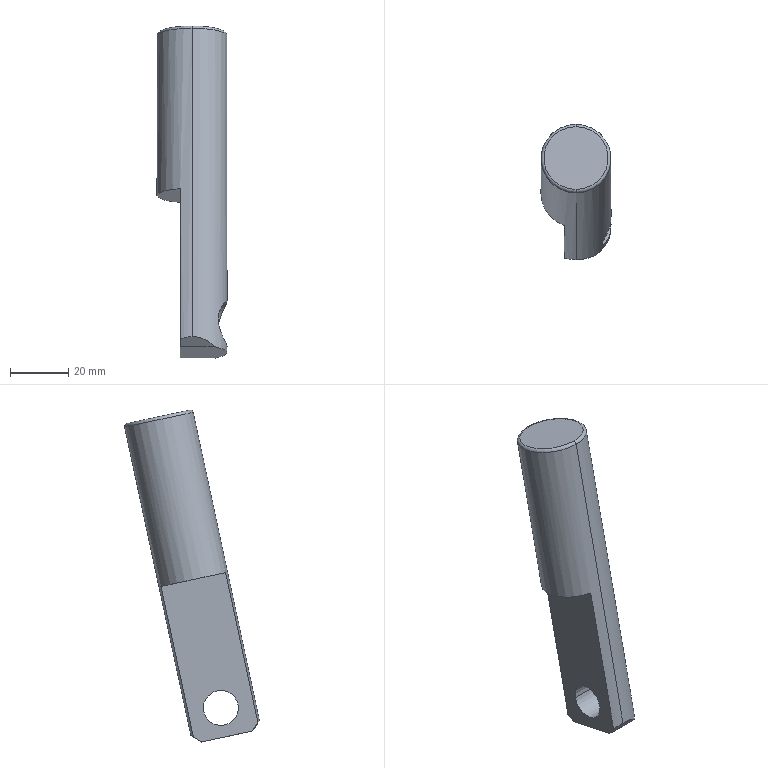Component | SolidWorks | SwingRod-2 | 1 solid | 15 faces | box 24 x 46.18 x 113.72 mm | volume 41126 mm3 | plane 7 | cylinder 6 | torus 2 | commonest cylinder face diameters 16 x2 12 x2 24 x2
STEP:
#1=COLOUR_RGB('',0.7922,0.8196,0.9333);
#2=FILL_AREA_STYLE_COLOUR('',#1);
#3=FILL_AREA_STYLE('',(#2));
#4=SURFACE_STYLE_FILL_AREA(#3);
#5=SURFACE_SIDE_STYLE('',(#4));
#6=SURFACE_STYLE_USAGE(.BOTH.,#5);
#7=PRESENTATION_STYLE_ASSIGNMENT((#6));
#8=CARTESIAN_POINT('',(6.39,3.505,17.411));
#9=VERTEX_POINT('',#8);
#10=CARTESIAN_POINT('',(6.39,2.658,17.593));
#11=VERTEX_POINT('',#10);
#12=CARTESIAN_POINT('',(6.39,3.081,17.502));
#13=DIRECTION('',(0.,0.2101,0.9777));
#14=DIRECTION('',(0.,-0.9777,0.2101));
#15=AXIS2_PLACEMENT_3D('',#12,#13,#14);
#16=CIRCLE('',#15,0.4331);
#17=EDGE_CURVE('',#9,#11,#16,.T.);
#18=ORIENTED_EDGE('',*,*,#17,.F.);
#19=CARTESIAN_POINT('',(6.39,3.535,17.365));
#20=VERTEX_POINT('',#19);
#21=CARTESIAN_POINT('',(6.39,3.496,17.373));
#22=DIRECTION('',(-1.,0.,0.));
#23=DIRECTION('',(0.,0.,1.));
#24=AXIS2_PLACEMENT_3D('',#21,#22,#23);
#25=CIRCLE('',#24,0.03937);
#26=EDGE_CURVE('',#9,#20,#25,.T.);
#27=ORIENTED_EDGE('',*,*,#26,.T.);
#28=CARTESIAN_POINT('',(6.39,2.611,17.563));
#29=VERTEX_POINT('',#28);
#30=CARTESIAN_POINT('',(6.39,3.073,17.464));
#31=DIRECTION('',(-0.,-0.2101,-0.9777));
#32=DIRECTION('',(0.,-0.9777,0.2101));
#33=AXIS2_PLACEMENT_3D('',#30,#31,#32);
#34=CIRCLE('',#33,0.4724);
#35=EDGE_CURVE('',#29,#20,#34,.T.);
#36=ORIENTED_EDGE('',*,*,#35,.F.);
#37=CARTESIAN_POINT('',(6.39,2.65,17.555));
#38=DIRECTION('',(1.,-0.,-0.));
#39=DIRECTION('',(-0.,0.,-1.));
#40=AXIS2_PLACEMENT_3D('',#37,#38,#39);
#41=CIRCLE('',#40,0.03937);
#42=EDGE_CURVE('',#11,#29,#41,.T.);
#43=ORIENTED_EDGE('',*,*,#42,.F.);
#44=EDGE_LOOP('',(#18,#27,#36,#43));
#45=FACE_OUTER_BOUND('',#44,.T.);
#46=CARTESIAN_POINT('',(6.39,3.073,17.464));
#47=DIRECTION('',(-0.,-0.2101,-0.9777));
#48=DIRECTION('',(0.,-0.9777,0.2101));
#49=AXIS2_PLACEMENT_3D('',#46,#47,#48);
#50=TOROIDAL_SURFACE('',#49,0.4331,0.03937);
#51=ADVANCED_FACE('',(#45),#50,.T.);
#52=CARTESIAN_POINT('',(6.742,2.546,13.51));
#53=VERTEX_POINT('',#52);
#54=CARTESIAN_POINT('',(6.742,1.93,13.642));
#55=VERTEX_POINT('',#54);
#56=CARTESIAN_POINT('',(6.742,2.546,13.51));
#57=CARTESIAN_POINT('',(6.742,2.55,13.531));
#58=CARTESIAN_POINT('',(6.744,2.552,13.552));
#59=CARTESIAN_POINT('',(6.749,2.553,13.584));
#60=CARTESIAN_POINT('',(6.751,2.552,13.594));
#61=CARTESIAN_POINT('',(6.757,2.55,13.615));
#62=CARTESIAN_POINT('',(6.759,2.549,13.625));
#63=CARTESIAN_POINT('',(6.766,2.545,13.645));
#64=CARTESIAN_POINT('',(6.769,2.543,13.655));
#65=CARTESIAN_POINT('',(6.776,2.537,13.674));
#66=CARTESIAN_POINT('',(6.779,2.534,13.684));
#67=CARTESIAN_POINT('',(6.791,2.523,13.712));
#68=CARTESIAN_POINT('',(6.798,2.514,13.73));
#69=CARTESIAN_POINT('',(6.813,2.492,13.763));
#70=CARTESIAN_POINT('',(6.821,2.479,13.779));
#71=CARTESIAN_POINT('',(6.834,2.452,13.808));
#72=CARTESIAN_POINT('',(6.84,2.436,13.822));
#73=CARTESIAN_POINT('',(6.848,2.411,13.839));
#74=CARTESIAN_POINT('',(6.85,2.402,13.845));
#75=CARTESIAN_POINT('',(6.855,2.384,13.855));
#76=CARTESIAN_POINT('',(6.856,2.375,13.86));
#77=CARTESIAN_POINT('',(6.861,2.346,13.873));
#78=CARTESIAN_POINT('',(6.862,2.326,13.88));
#79=CARTESIAN_POINT('',(6.862,2.294,13.886));
#80=CARTESIAN_POINT('',(6.862,2.284,13.888));
#81=CARTESIAN_POINT('',(6.86,2.262,13.89));
#82=CARTESIAN_POINT('',(6.859,2.252,13.891));
#83=CARTESIAN_POINT('',(6.855,2.22,13.891));
#84=CARTESIAN_POINT('',(6.851,2.199,13.89));
#85=CARTESIAN_POINT('',(6.841,2.158,13.882));
#86=CARTESIAN_POINT('',(6.835,2.138,13.876));
#87=CARTESIAN_POINT('',(6.821,2.101,13.861));
#88=CARTESIAN_POINT('',(6.814,2.083,13.851));
#89=CARTESIAN_POINT('',(6.798,2.049,13.83));
#90=CARTESIAN_POINT('',(6.791,2.034,13.817));
#91=CARTESIAN_POINT('',(6.776,2.005,13.789));
#92=CARTESIAN_POINT('',(6.769,1.992,13.774));
#93=CARTESIAN_POINT('',(6.76,1.974,13.749));
#94=CARTESIAN_POINT('',(6.757,1.969,13.74));
#95=CARTESIAN_POINT('',(6.751,1.958,13.722));
#96=CARTESIAN_POINT('',(6.749,1.954,13.713));
#97=CARTESIAN_POINT('',(6.746,1.945,13.694));
#98=CARTESIAN_POINT('',(6.744,1.941,13.684));
#99=CARTESIAN_POINT('',(6.742,1.935,13.663));
#100=CARTESIAN_POINT('',(6.742,1.932,13.653));
#101=CARTESIAN_POINT('',(6.742,1.93,13.642));
#102=B_SPLINE_CURVE_WITH_KNOTS('',3,(#56,#57,#58,#59,#60,#61,#62,#63,#64,#65,#66,#67,#68,#69,#70,#71,#72,#73,#74,#75,#76,#77,#78,#79,#80,#81,#82,#83,#84,#85,#86,#87,#88,#89,#90,#91,#92,#93,#94,#95,#96,#97,#98,#99,#100,#101),.UNSPECIFIED.,.F.,.F.,(4,2,2,2,2,2,2,2,2,2,2,2,2,2,2,2,2,2,2,2,2,2,4),(0.,0.001615,0.002422,0.00323,0.004037,0.004845,0.00646,0.008075,0.00969,0.0105,0.0113,0.01292,0.01373,0.01453,0.01615,0.01776,0.01938,0.02099,0.02261,0.02342,0.02422,0.02503,0.02584),.UNSPECIFIED.);
#103=EDGE_CURVE('',#53,#55,#102,.T.);
#104=ORIENTED_EDGE('',*,*,#103,.T.);
#105=CARTESIAN_POINT('',(6.626,1.93,13.642));
#106=VERTEX_POINT('',#105);
#107=CARTESIAN_POINT('',(6.862,1.93,13.642));
#108=DIRECTION('',(-1.,0.,0.));
#109=VECTOR('',#108,39.37);
#110=LINE('',#107,#109);
#111=EDGE_CURVE('',#55,#106,#110,.T.);
#112=ORIENTED_EDGE('',*,*,#111,.T.);
#113=CARTESIAN_POINT('',(6.626,2.546,13.51));
#114=VERTEX_POINT('',#113);
#115=CARTESIAN_POINT('',(6.626,2.238,13.576));
#116=DIRECTION('',(-1.,0.,0.));
#117=DIRECTION('',(-0.,0.9777,-0.2101));
#118=AXIS2_PLACEMENT_3D('',#115,#116,#117);
#119=CIRCLE('',#118,0.315);
#120=EDGE_CURVE('',#106,#114,#119,.T.);
#121=ORIENTED_EDGE('',*,*,#120,.T.);
#122=CARTESIAN_POINT('',(6.862,2.546,13.51));
#123=DIRECTION('',(-1.,0.,0.));
#124=VECTOR('',#123,39.37);
#125=LINE('',#122,#124);
#126=EDGE_CURVE('',#53,#114,#125,.T.);
#127=ORIENTED_EDGE('',*,*,#126,.F.);
#128=EDGE_LOOP('',(#104,#112,#121,#127));
#129=FACE_OUTER_BOUND('',#128,.T.);
#130=CARTESIAN_POINT('',(6.862,2.238,13.576));
#131=DIRECTION('',(-1.,0.,0.));
#132=DIRECTION('',(-0.,0.9777,-0.2101));
#133=AXIS2_PLACEMENT_3D('',#130,#131,#132);
#134=CYLINDRICAL_SURFACE('',#133,0.315);
#135=ADVANCED_FACE('',(#129),#134,.F.);
#136=CARTESIAN_POINT('',(6.626,2.007,13.626));
#137=VERTEX_POINT('',#136);
#138=CARTESIAN_POINT('',(6.626,2.469,13.527));
#139=VERTEX_POINT('',#138);
#140=CARTESIAN_POINT('',(6.626,2.238,13.576));
#141=DIRECTION('',(-1.,0.,0.));
#142=DIRECTION('',(-0.,0.9777,-0.2101));
#143=AXIS2_PLACEMENT_3D('',#140,#141,#142);
#144=CIRCLE('',#143,0.2362);
#145=EDGE_CURVE('',#137,#139,#144,.T.);
#146=ORIENTED_EDGE('',*,*,#145,.F.);
#147=CARTESIAN_POINT('',(6.232,2.007,13.626));
#148=VERTEX_POINT('',#147);
#149=CARTESIAN_POINT('',(6.626,2.007,13.626));
#150=DIRECTION('',(-1.,0.,0.));
#151=VECTOR('',#150,39.37);
#152=LINE('',#149,#151);
#153=EDGE_CURVE('',#137,#148,#152,.T.);
#154=ORIENTED_EDGE('',*,*,#153,.T.);
#155=CARTESIAN_POINT('',(6.232,2.469,13.527));
#156=VERTEX_POINT('',#155);
#157=CARTESIAN_POINT('',(6.232,2.238,13.576));
#158=DIRECTION('',(-1.,0.,0.));
#159=DIRECTION('',(-0.,0.9777,-0.2101));
#160=AXIS2_PLACEMENT_3D('',#157,#158,#159);
#161=CIRCLE('',#160,0.2362);
#162=EDGE_CURVE('',#148,#156,#161,.T.);
#163=ORIENTED_EDGE('',*,*,#162,.T.);
#164=CARTESIAN_POINT('',(6.626,2.469,13.527));
#165=DIRECTION('',(-1.,0.,0.));
#166=VECTOR('',#165,39.37);
#167=LINE('',#164,#166);
#168=EDGE_CURVE('',#139,#156,#167,.T.);
#169=ORIENTED_EDGE('',*,*,#168,.F.);
#170=EDGE_LOOP('',(#146,#154,#163,#169));
#171=FACE_OUTER_BOUND('',#170,.T.);
#172=CARTESIAN_POINT('',(6.626,2.238,13.576));
#173=DIRECTION('',(-1.,0.,0.));
#174=DIRECTION('',(-0.,0.9777,-0.2101));
#175=AXIS2_PLACEMENT_3D('',#172,#173,#174);
#176=CYLINDRICAL_SURFACE('',#175,0.2362);
#177=ADVANCED_FACE('',(#171),#176,.F.);
#178=CARTESIAN_POINT('',(6.232,1.739,13.374));
#179=VERTEX_POINT('',#178);
#180=CARTESIAN_POINT('',(6.39,1.718,13.406));
#181=VERTEX_POINT('',#180);
#182=CARTESIAN_POINT('',(6.232,1.739,13.374));
#183=CARTESIAN_POINT('',(6.283,1.725,13.395));
#184=CARTESIAN_POINT('',(6.336,1.718,13.406));
#185=CARTESIAN_POINT('',(6.39,1.718,13.406));
#186=(BOUNDED_CURVE()B_SPLINE_CURVE(3,(#182,#183,#184,#185),.UNSPECIFIED.,.F.,.F.)B_SPLINE_CURVE_WITH_KNOTS((4,4),(5.943,6.283),.UNSPECIFIED.)CURVE()GEOMETRIC_REPRESENTATION_ITEM()RATIONAL_B_SPLINE_CURVE((1.,0.9904,0.9904,1.))REPRESENTATION_ITEM(''));
#187=EDGE_CURVE('',#179,#181,#186,.T.);
#188=ORIENTED_EDGE('',*,*,#187,.T.);
#189=CARTESIAN_POINT('',(6.39,1.693,13.291));
#190=DIRECTION('',(0.,0.2101,0.9777));
#191=VECTOR('',#190,39.37);
#192=LINE('',#189,#191);
#193=EDGE_CURVE('',#181,#29,#192,.T.);
#194=ORIENTED_EDGE('',*,*,#193,.T.);
#195=ORIENTED_EDGE('',*,*,#35,.T.);
#196=CARTESIAN_POINT('',(6.39,2.642,13.208));
#197=VERTEX_POINT('',#196);
#198=CARTESIAN_POINT('',(6.39,2.617,13.092));
#199=DIRECTION('',(0.,0.2101,0.9777));
#200=VECTOR('',#199,39.37);
#201=LINE('',#198,#200);
#202=EDGE_CURVE('',#197,#20,#201,.T.);
#203=ORIENTED_EDGE('',*,*,#202,.F.);
#204=CARTESIAN_POINT('',(6.232,2.61,13.187));
#205=VERTEX_POINT('',#204);
#206=CARTESIAN_POINT('',(6.39,2.642,13.208));
#207=CARTESIAN_POINT('',(6.336,2.642,13.208));
#208=CARTESIAN_POINT('',(6.283,2.631,13.201));
#209=CARTESIAN_POINT('',(6.232,2.61,13.187));
#210=(BOUNDED_CURVE()B_SPLINE_CURVE(3,(#206,#207,#208,#209),.UNSPECIFIED.,.F.,.F.)B_SPLINE_CURVE_WITH_KNOTS((4,4),(0.,0.3398),.UNSPECIFIED.)CURVE()GEOMETRIC_REPRESENTATION_ITEM()RATIONAL_B_SPLINE_CURVE((1.,0.9904,0.9904,1.))REPRESENTATION_ITEM(''));
#211=EDGE_CURVE('',#197,#205,#210,.T.);
#212=ORIENTED_EDGE('',*,*,#211,.T.);
#213=CARTESIAN_POINT('',(6.232,3.045,15.215));
#214=VERTEX_POINT('',#213);
#215=CARTESIAN_POINT('',(6.232,3.045,15.215));
#216=DIRECTION('',(-0.,-0.2101,-0.9777));
#217=VECTOR('',#216,39.37);
#218=LINE('',#215,#217);
#219=EDGE_CURVE('',#214,#205,#218,.T.);
#220=ORIENTED_EDGE('',*,*,#219,.F.);
#221=CARTESIAN_POINT('',(6.232,2.174,15.402));
#222=VERTEX_POINT('',#221);
#223=CARTESIAN_POINT('',(6.39,2.61,15.308));
#224=DIRECTION('',(-0.,-0.2101,-0.9777));
#225=DIRECTION('',(0.,-0.9777,0.2101));
#226=AXIS2_PLACEMENT_3D('',#223,#224,#225);
#227=CIRCLE('',#226,0.4724);
#228=EDGE_CURVE('',#222,#214,#227,.T.);
#229=ORIENTED_EDGE('',*,*,#228,.F.);
#230=CARTESIAN_POINT('',(6.232,2.174,15.402));
#231=DIRECTION('',(-0.,-0.2101,-0.9777));
#232=VECTOR('',#231,39.37);
#233=LINE('',#230,#232);
#234=EDGE_CURVE('',#222,#179,#233,.T.);
#235=ORIENTED_EDGE('',*,*,#234,.T.);
#236=EDGE_LOOP('',(#188,#194,#195,#203,#212,#220,#229,#235));
#237=FACE_OUTER_BOUND('',#236,.T.);
#238=CARTESIAN_POINT('',(6.39,2.155,13.191));
#239=DIRECTION('',(0.,0.2101,0.9777));
#240=DIRECTION('',(-0.,0.9777,-0.2101));
#241=AXIS2_PLACEMENT_3D('',#238,#239,#240);
#242=CYLINDRICAL_SURFACE('',#241,0.4724);
#243=ADVANCED_FACE('',(#237),#242,.T.);
#244=ORIENTED_EDGE('',*,*,#193,.F.);
#245=CARTESIAN_POINT('',(6.702,1.809,13.266));
#246=VERTEX_POINT('',#245);
#247=CARTESIAN_POINT('',(6.39,1.718,13.406));
#248=CARTESIAN_POINT('',(6.506,1.718,13.406));
#249=CARTESIAN_POINT('',(6.615,1.749,13.357));
#250=CARTESIAN_POINT('',(6.702,1.809,13.266));
#251=(BOUNDED_CURVE()B_SPLINE_CURVE(3,(#247,#248,#249,#250),.UNSPECIFIED.,.F.,.F.)B_SPLINE_CURVE_WITH_KNOTS((4,4),(0.,0.7227),.UNSPECIFIED.)CURVE()GEOMETRIC_REPRESENTATION_ITEM()RATIONAL_B_SPLINE_CURVE((1.,0.9569,0.9569,1.))REPRESENTATION_ITEM(''));
#252=EDGE_CURVE('',#181,#246,#251,.T.);
#253=ORIENTED_EDGE('',*,*,#252,.T.);
#254=CARTESIAN_POINT('',(6.702,2.501,13.117));
#255=VERTEX_POINT('',#254);
#256=CARTESIAN_POINT('',(6.39,2.155,13.191));
#257=DIRECTION('',(-0.,-0.2101,-0.9777));
#258=DIRECTION('',(0.,-0.9777,0.2101));
#259=AXIS2_PLACEMENT_3D('',#256,#257,#258);
#260=CIRCLE('',#259,0.4724);
#261=EDGE_CURVE('',#255,#246,#260,.T.);
#262=ORIENTED_EDGE('',*,*,#261,.F.);
#263=CARTESIAN_POINT('',(6.702,2.501,13.117));
#264=CARTESIAN_POINT('',(6.615,2.593,13.176));
#265=CARTESIAN_POINT('',(6.506,2.642,13.208));
#266=CARTESIAN_POINT('',(6.39,2.642,13.208));
#267=(BOUNDED_CURVE()B_SPLINE_CURVE(3,(#263,#264,#265,#266),.UNSPECIFIED.,.F.,.F.)B_SPLINE_CURVE_WITH_KNOTS((4,4),(5.56,6.283),.UNSPECIFIED.)CURVE()GEOMETRIC_REPRESENTATION_ITEM()RATIONAL_B_SPLINE_CURVE((1.,0.9569,0.9569,1.))REPRESENTATION_ITEM(''));
#268=EDGE_CURVE('',#255,#197,#267,.T.);
#269=ORIENTED_EDGE('',*,*,#268,.T.);
#270=ORIENTED_EDGE('',*,*,#202,.T.);
#271=CARTESIAN_POINT('',(6.39,3.073,17.464));
#272=DIRECTION('',(-0.,-0.2101,-0.9777));
#273=DIRECTION('',(0.,-0.9777,0.2101));
#274=AXIS2_PLACEMENT_3D('',#271,#272,#273);
#275=CIRCLE('',#274,0.4724);
#276=EDGE_CURVE('',#20,#29,#275,.T.);
#277=ORIENTED_EDGE('',*,*,#276,.T.);
#278=EDGE_LOOP('',(#244,#253,#262,#269,#270,#277));
#279=FACE_OUTER_BOUND('',#278,.T.);
#280=ORIENTED_EDGE('',*,*,#103,.F.);
#281=CARTESIAN_POINT('',(6.742,1.93,13.642));
#282=CARTESIAN_POINT('',(6.742,1.925,13.622));
#283=CARTESIAN_POINT('',(6.744,1.923,13.601));
#284=CARTESIAN_POINT('',(6.751,1.923,13.558));
#285=CARTESIAN_POINT('',(6.756,1.924,13.538));
#286=CARTESIAN_POINT('',(6.766,1.93,13.507));
#287=CARTESIAN_POINT('',(6.769,1.933,13.497));
#288=CARTESIAN_POINT('',(6.776,1.938,13.478));
#289=CARTESIAN_POINT('',(6.779,1.942,13.469));
#290=CARTESIAN_POINT('',(6.787,1.949,13.45));
#291=CARTESIAN_POINT('',(6.791,1.953,13.441));
#292=CARTESIAN_POINT('',(6.798,1.962,13.423));
#293=CARTESIAN_POINT('',(6.802,1.967,13.415));
#294=CARTESIAN_POINT('',(6.813,1.983,13.389));
#295=CARTESIAN_POINT('',(6.821,1.996,13.374));
#296=CARTESIAN_POINT('',(6.831,2.017,13.352));
#297=CARTESIAN_POINT('',(6.834,2.024,13.345));
#298=CARTESIAN_POINT('',(6.84,2.039,13.331));
#299=CARTESIAN_POINT('',(6.843,2.048,13.325));
#300=CARTESIAN_POINT('',(6.851,2.073,13.307));
#301=CARTESIAN_POINT('',(6.855,2.091,13.297));
#302=CARTESIAN_POINT('',(6.859,2.12,13.284));
#303=CARTESIAN_POINT('',(6.86,2.13,13.28));
#304=CARTESIAN_POINT('',(6.862,2.151,13.273));
#305=CARTESIAN_POINT('',(6.862,2.161,13.271));
#306=CARTESIAN_POINT('',(6.862,2.182,13.266));
#307=CARTESIAN_POINT('',(6.862,2.192,13.265));
#308=CARTESIAN_POINT('',(6.86,2.213,13.262));
#309=CARTESIAN_POINT('',(6.859,2.224,13.261));
#310=CARTESIAN_POINT('',(6.855,2.256,13.261));
#311=CARTESIAN_POINT('',(6.851,2.277,13.263));
#312=CARTESIAN_POINT('',(6.841,2.318,13.271));
#313=CARTESIAN_POINT('',(6.834,2.337,13.277));
#314=CARTESIAN_POINT('',(6.821,2.375,13.292));
#315=CARTESIAN_POINT('',(6.813,2.393,13.301));
#316=CARTESIAN_POINT('',(6.798,2.426,13.323));
#317=CARTESIAN_POINT('',(6.791,2.442,13.335));
#318=CARTESIAN_POINT('',(6.78,2.463,13.356));
#319=CARTESIAN_POINT('',(6.776,2.47,13.364));
#320=CARTESIAN_POINT('',(6.769,2.483,13.379));
#321=CARTESIAN_POINT('',(6.766,2.49,13.387));
#322=CARTESIAN_POINT('',(6.759,2.501,13.404));
#323=CARTESIAN_POINT('',(6.757,2.507,13.412));
#324=CARTESIAN_POINT('',(6.751,2.517,13.43));
#325=CARTESIAN_POINT('',(6.749,2.522,13.44));
#326=CARTESIAN_POINT('',(6.744,2.534,13.469));
#327=CARTESIAN_POINT('',(6.742,2.541,13.489));
#328=CARTESIAN_POINT('',(6.742,2.546,13.51));
#329=B_SPLINE_CURVE_WITH_KNOTS('',3,(#281,#282,#283,#284,#285,#286,#287,#288,#289,#290,#291,#292,#293,#294,#295,#296,#297,#298,#299,#300,#301,#302,#303,#304,#305,#306,#307,#308,#309,#310,#311,#312,#313,#314,#315,#316,#317,#318,#319,#320,#321,#322,#323,#324,#325,#326,#327,#328),.UNSPECIFIED.,.F.,.F.,(4,2,2,2,2,2,2,2,2,2,2,2,2,2,2,2,2,2,2,2,2,2,2,4),(0.02584,0.02745,0.02906,0.02986,0.03067,0.03147,0.03228,0.03389,0.03469,0.0355,0.03711,0.03791,0.03872,0.03952,0.04033,0.04194,0.04355,0.04516,0.04677,0.04757,0.04838,0.04919,0.04999,0.0516),.UNSPECIFIED.);
#330=EDGE_CURVE('',#55,#53,#329,.T.);
#331=ORIENTED_EDGE('',*,*,#330,.F.);
#332=EDGE_LOOP('',(#280,#331));
#333=FACE_BOUND('',#332,.T.);
#334=CARTESIAN_POINT('',(6.39,2.155,13.191));
#335=DIRECTION('',(0.,0.2101,0.9777));
#336=DIRECTION('',(-0.,0.9777,-0.2101));
#337=AXIS2_PLACEMENT_3D('',#334,#335,#336);
#338=CYLINDRICAL_SURFACE('',#337,0.4724);
#339=ADVANCED_FACE('',(#279,#333),#338,.T.);
#340=ORIENTED_EDGE('',*,*,#261,.T.);
#341=CARTESIAN_POINT('',(6.232,1.809,13.266));
#342=VERTEX_POINT('',#341);
#343=CARTESIAN_POINT('',(6.862,1.809,13.266));
#344=DIRECTION('',(-1.,0.,0.));
#345=VECTOR('',#344,39.37);
#346=LINE('',#343,#345);
#347=EDGE_CURVE('',#246,#342,#346,.T.);
#348=ORIENTED_EDGE('',*,*,#347,.T.);
#349=CARTESIAN_POINT('',(6.232,2.501,13.117));
#350=VERTEX_POINT('',#349);
#351=CARTESIAN_POINT('',(6.232,2.155,13.191));
#352=DIRECTION('',(0.,-0.9777,0.2101));
#353=VECTOR('',#352,39.37);
#354=LINE('',#351,#353);
#355=EDGE_CURVE('',#350,#342,#354,.T.);
#356=ORIENTED_EDGE('',*,*,#355,.F.);
#357=CARTESIAN_POINT('',(6.862,2.501,13.117));
#358=DIRECTION('',(-1.,0.,0.));
#359=VECTOR('',#358,39.37);
#360=LINE('',#357,#359);
#361=EDGE_CURVE('',#255,#350,#360,.T.);
#362=ORIENTED_EDGE('',*,*,#361,.F.);
#363=EDGE_LOOP('',(#340,#348,#356,#362));
#364=FACE_OUTER_BOUND('',#363,.T.);
#365=CARTESIAN_POINT('',(6.39,2.155,13.191));
#366=DIRECTION('',(-0.,-0.2101,-0.9777));
#367=DIRECTION('',(0.,-0.9777,0.2101));
#368=AXIS2_PLACEMENT_3D('',#365,#366,#367);
#369=PLANE('',#368);
#370=ADVANCED_FACE('',(#364),#369,.T.);
#371=CARTESIAN_POINT('',(6.232,2.238,13.576));
#372=DIRECTION('',(-1.,0.,0.));
#373=DIRECTION('',(-0.,0.9777,-0.2101));
#374=AXIS2_PLACEMENT_3D('',#371,#372,#373);
#375=CIRCLE('',#374,0.2362);
#376=EDGE_CURVE('',#156,#148,#375,.T.);
#377=ORIENTED_EDGE('',*,*,#376,.F.);
#378=ORIENTED_EDGE('',*,*,#162,.F.);
#379=EDGE_LOOP('',(#377,#378));
#380=FACE_BOUND('',#379,.T.);
#381=CARTESIAN_POINT('',(6.232,0.2522,15.674));
#382=DIRECTION('',(0.,-0.5428,0.8399));
#383=VECTOR('',#382,39.37);
#384=LINE('',#381,#383);
#385=EDGE_CURVE('',#342,#179,#384,.T.);
#386=ORIENTED_EDGE('',*,*,#385,.T.);
#387=ORIENTED_EDGE('',*,*,#234,.F.);
#388=CARTESIAN_POINT('',(6.232,2.61,15.308));
#389=DIRECTION('',(0.,-0.9777,0.2101));
#390=VECTOR('',#389,39.37);
#391=LINE('',#388,#390);
#392=EDGE_CURVE('',#214,#222,#391,.T.);
#393=ORIENTED_EDGE('',*,*,#392,.F.);
#394=ORIENTED_EDGE('',*,*,#219,.T.);
#395=CARTESIAN_POINT('',(6.232,4.91,14.673));
#396=DIRECTION('',(-0.,-0.8399,-0.5428));
#397=VECTOR('',#396,39.37);
#398=LINE('',#395,#397);
#399=EDGE_CURVE('',#205,#350,#398,.T.);
#400=ORIENTED_EDGE('',*,*,#399,.T.);
#401=ORIENTED_EDGE('',*,*,#355,.T.);
#402=EDGE_LOOP('',(#386,#387,#393,#394,#400,#401));
#403=FACE_OUTER_BOUND('',#402,.T.);
#404=CARTESIAN_POINT('',(6.232,2.61,15.308));
#405=DIRECTION('',(1.,-0.,-0.));
#406=DIRECTION('',(0.,-0.9777,0.2101));
#407=AXIS2_PLACEMENT_3D('',#404,#405,#406);
#408=PLANE('',#407);
#409=ADVANCED_FACE('',(#380,#403),#408,.F.);
#410=CARTESIAN_POINT('',(6.39,3.081,17.502));
#411=DIRECTION('',(0.,0.2101,0.9777));
#412=DIRECTION('',(0.,-0.9777,0.2101));
#413=AXIS2_PLACEMENT_3D('',#410,#411,#412);
#414=CIRCLE('',#413,0.4331);
#415=EDGE_CURVE('',#11,#9,#414,.T.);
#416=ORIENTED_EDGE('',*,*,#415,.T.);
#417=ORIENTED_EDGE('',*,*,#17,.T.);
#418=EDGE_LOOP('',(#416,#417));
#419=FACE_OUTER_BOUND('',#418,.T.);
#420=CARTESIAN_POINT('',(6.39,3.081,17.502));
#421=DIRECTION('',(-0.,-0.2101,-0.9777));
#422=DIRECTION('',(0.,-0.9777,0.2101));
#423=AXIS2_PLACEMENT_3D('',#420,#421,#422);
#424=PLANE('',#423);
#425=ADVANCED_FACE('',(#419),#424,.F.);
#426=ORIENTED_EDGE('',*,*,#228,.T.);
#427=ORIENTED_EDGE('',*,*,#392,.T.);
#428=EDGE_LOOP('',(#426,#427));
#429=FACE_OUTER_BOUND('',#428,.T.);
#430=CARTESIAN_POINT('',(6.39,2.61,15.308));
#431=DIRECTION('',(-0.,-0.2101,-0.9777));
#432=DIRECTION('',(0.,-0.9777,0.2101));
#433=AXIS2_PLACEMENT_3D('',#430,#431,#432);
#434=PLANE('',#433);
#435=ADVANCED_FACE('',(#429),#434,.T.);
#436=ORIENTED_EDGE('',*,*,#153,.F.);
#437=CARTESIAN_POINT('',(6.626,2.238,13.576));
#438=DIRECTION('',(-1.,0.,0.));
#439=DIRECTION('',(-0.,0.9777,-0.2101));
#440=AXIS2_PLACEMENT_3D('',#437,#438,#439);
#441=CIRCLE('',#440,0.2362);
#442=EDGE_CURVE('',#139,#137,#441,.T.);
#443=ORIENTED_EDGE('',*,*,#442,.F.);
#444=ORIENTED_EDGE('',*,*,#168,.T.);
#445=ORIENTED_EDGE('',*,*,#376,.T.);
#446=EDGE_LOOP('',(#436,#443,#444,#445));
#447=FACE_OUTER_BOUND('',#446,.T.);
#448=CARTESIAN_POINT('',(6.626,2.238,13.576));
#449=DIRECTION('',(-1.,0.,0.));
#450=DIRECTION('',(-0.,0.9777,-0.2101));
#451=AXIS2_PLACEMENT_3D('',#448,#449,#450);
#452=CYLINDRICAL_SURFACE('',#451,0.2362);
#453=ADVANCED_FACE('',(#447),#452,.F.);
#454=ORIENTED_EDGE('',*,*,#111,.F.);
#455=ORIENTED_EDGE('',*,*,#330,.T.);
#456=ORIENTED_EDGE('',*,*,#126,.T.);
#457=CARTESIAN_POINT('',(6.626,2.238,13.576));
#458=DIRECTION('',(-1.,0.,0.));
#459=DIRECTION('',(-0.,0.9777,-0.2101));
#460=AXIS2_PLACEMENT_3D('',#457,#458,#459);
#461=CIRCLE('',#460,0.315);
#462=EDGE_CURVE('',#114,#106,#461,.T.);
#463=ORIENTED_EDGE('',*,*,#462,.T.);
#464=EDGE_LOOP('',(#454,#455,#456,#463));
#465=FACE_OUTER_BOUND('',#464,.T.);
#466=CARTESIAN_POINT('',(6.862,2.238,13.576));
#467=DIRECTION('',(-1.,0.,0.));
#468=DIRECTION('',(-0.,0.9777,-0.2101));
#469=AXIS2_PLACEMENT_3D('',#466,#467,#468);
#470=CYLINDRICAL_SURFACE('',#469,0.315);
#471=ADVANCED_FACE('',(#465),#470,.F.);
#472=ORIENTED_EDGE('',*,*,#442,.T.);
#473=ORIENTED_EDGE('',*,*,#145,.T.);
#474=EDGE_LOOP('',(#472,#473));
#475=FACE_BOUND('',#474,.T.);
#476=ORIENTED_EDGE('',*,*,#462,.F.);
#477=ORIENTED_EDGE('',*,*,#120,.F.);
#478=EDGE_LOOP('',(#476,#477));
#479=FACE_OUTER_BOUND('',#478,.T.);
#480=CARTESIAN_POINT('',(6.626,2.238,13.576));
#481=DIRECTION('',(-1.,0.,0.));
#482=DIRECTION('',(-0.,0.9777,-0.2101));
#483=AXIS2_PLACEMENT_3D('',#480,#481,#482);
#484=PLANE('',#483);
#485=ADVANCED_FACE('',(#475,#479),#484,.F.);
#486=ORIENTED_EDGE('',*,*,#268,.F.);
#487=ORIENTED_EDGE('',*,*,#361,.T.);
#488=ORIENTED_EDGE('',*,*,#399,.F.);
#489=ORIENTED_EDGE('',*,*,#211,.F.);
#490=EDGE_LOOP('',(#486,#487,#488,#489));
#491=FACE_OUTER_BOUND('',#490,.T.);
#492=CARTESIAN_POINT('',(6.862,4.91,14.673));
#493=DIRECTION('',(-0.,0.5428,-0.8399));
#494=DIRECTION('',(-0.,-0.8399,-0.5428));
#495=AXIS2_PLACEMENT_3D('',#492,#493,#494);
#496=PLANE('',#495);
#497=ADVANCED_FACE('',(#491),#496,.T.);
#498=ORIENTED_EDGE('',*,*,#187,.F.);
#499=ORIENTED_EDGE('',*,*,#385,.F.);
#500=ORIENTED_EDGE('',*,*,#347,.F.);
#501=ORIENTED_EDGE('',*,*,#252,.F.);
#502=EDGE_LOOP('',(#498,#499,#500,#501));
#503=FACE_OUTER_BOUND('',#502,.T.);
#504=CARTESIAN_POINT('',(6.862,0.2522,15.674));
#505=DIRECTION('',(-0.,-0.8399,-0.5428));
#506=DIRECTION('',(0.,-0.5428,0.8399));
#507=AXIS2_PLACEMENT_3D('',#504,#505,#506);
#508=PLANE('',#507);
#509=ADVANCED_FACE('',(#503),#508,.T.);
#510=ORIENTED_EDGE('',*,*,#26,.F.);
#511=ORIENTED_EDGE('',*,*,#415,.F.);
#512=ORIENTED_EDGE('',*,*,#42,.T.);
#513=ORIENTED_EDGE('',*,*,#276,.F.);
#514=EDGE_LOOP('',(#510,#511,#512,#513));
#515=FACE_OUTER_BOUND('',#514,.T.);
#516=CARTESIAN_POINT('',(6.39,3.073,17.464));
#517=DIRECTION('',(-0.,-0.2101,-0.9777));
#518=DIRECTION('',(0.,-0.9777,0.2101));
#519=AXIS2_PLACEMENT_3D('',#516,#517,#518);
#520=TOROIDAL_SURFACE('',#519,0.4331,0.03937);
#521=ADVANCED_FACE('',(#515),#520,.T.);
#522=CLOSED_SHELL('',(#51,#135,#177,#243,#339,#370,#409,#425,#435,#453,#471,#485,#497,#509,#521));
#523=MANIFOLD_SOLID_BREP('',#522);
#524=STYLED_ITEM('',(#7),#523);
#525=PRESENTATION_LAYER_ASSIGNMENT('','',(#524));
#526=(LENGTH_UNIT()NAMED_UNIT(*)SI_UNIT($,.METRE.));
#527=LENGTH_MEASURE_WITH_UNIT(LENGTH_MEASURE(0.0254),#526);
#528=DIMENSIONAL_EXPONENTS(1.,0.,0.,0.,0.,0.,0.);
#529=(CONVERSION_BASED_UNIT('',#527)LENGTH_UNIT()NAMED_UNIT(#528));
#530=UNCERTAINTY_MEASURE_WITH_UNIT(LENGTH_MEASURE(0.00001),#529,'','');
#531=(NAMED_UNIT(*)PLANE_ANGLE_UNIT()SI_UNIT($,.RADIAN.));
#532=(NAMED_UNIT(*)SI_UNIT($,.STERADIAN.)SOLID_ANGLE_UNIT());
#533=(GEOMETRIC_REPRESENTATION_CONTEXT(3)GLOBAL_UNCERTAINTY_ASSIGNED_CONTEXT((#530))GLOBAL_UNIT_ASSIGNED_CONTEXT((#529,#531,#532))REPRESENTATION_CONTEXT('',''));
#534=MECHANICAL_DESIGN_GEOMETRIC_PRESENTATION_REPRESENTATION('',(#524),#533);
#535=CARTESIAN_POINT('',(0.,0.,0.));
#536=DIRECTION('',(0.,0.,1.));
#537=DIRECTION('',(1.,0.,0.));
#538=AXIS2_PLACEMENT_3D('',#535,#536,#537);
#539=(LENGTH_UNIT()NAMED_UNIT(*)SI_UNIT($,.METRE.));
#540=LENGTH_MEASURE_WITH_UNIT(LENGTH_MEASURE(0.0254),#539);
#541=DIMENSIONAL_EXPONENTS(1.,0.,0.,0.,0.,0.,0.);
#542=(CONVERSION_BASED_UNIT('',#540)LENGTH_UNIT()NAMED_UNIT(#541));
#543=UNCERTAINTY_MEASURE_WITH_UNIT(LENGTH_MEASURE(0.00001),#542,'','');
#544=(NAMED_UNIT(*)PLANE_ANGLE_UNIT()SI_UNIT($,.RADIAN.));
#545=(NAMED_UNIT(*)SI_UNIT($,.STERADIAN.)SOLID_ANGLE_UNIT());
#546=(GEOMETRIC_REPRESENTATION_CONTEXT(3)GLOBAL_UNCERTAINTY_ASSIGNED_CONTEXT((#543))GLOBAL_UNIT_ASSIGNED_CONTEXT((#542,#544,#545))REPRESENTATION_CONTEXT('',''));
#547=ADVANCED_BREP_SHAPE_REPRESENTATION('',(#523,#538),#546);